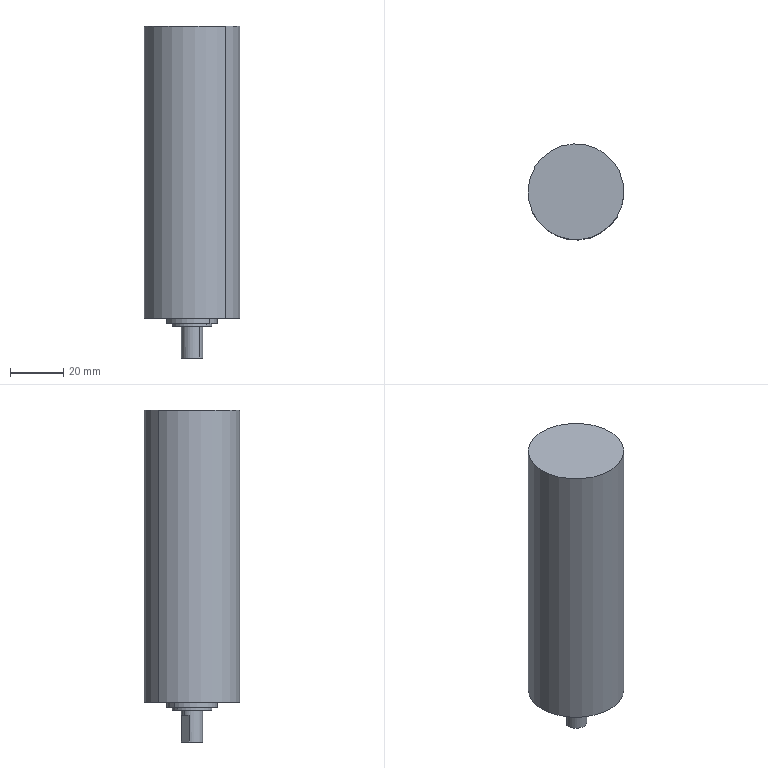Component | SolidWorks | MotorAssemblyWhen2-1_1.5KW-80-ER16A2-1 | 1 solid | 31 faces | box 36 x 36 x 124.7 mm | volume 112823 mm3 | cylinder 16 | cone 8 | plane 7 | commonest cylinder face diameters 2.5 x8 36 x2 19 x2 15 x2 8 x2
STEP:
#1=CARTESIAN_POINT('',(-1.467,4.834,0.5316));
#2=VERTEX_POINT('',#1);
#3=CARTESIAN_POINT('',(-2.47,5.836,0.5316));
#4=VERTEX_POINT('',#3);
#5=CARTESIAN_POINT('',(-1.969,5.335,0.5316));
#6=DIRECTION('',(-0.,0.,-1.));
#7=DIRECTION('',(0.7071,-0.7071,-0.));
#8=AXIS2_PLACEMENT_3D('',#5,#6,#7);
#9=CIRCLE('',#8,0.7087);
#10=EDGE_CURVE('',#2,#4,#9,.T.);
#11=ORIENTED_EDGE('',*,*,#10,.T.);
#12=CARTESIAN_POINT('',(-2.47,5.836,-3.787));
#13=VERTEX_POINT('',#12);
#14=CARTESIAN_POINT('',(-2.47,5.836,0.5316));
#15=DIRECTION('',(-0.,0.,-1.));
#16=VECTOR('',#15,39.37);
#17=LINE('',#14,#16);
#18=EDGE_CURVE('',#4,#13,#17,.T.);
#19=ORIENTED_EDGE('',*,*,#18,.T.);
#20=CARTESIAN_POINT('',(-1.467,4.834,-3.787));
#21=VERTEX_POINT('',#20);
#22=CARTESIAN_POINT('',(-1.969,5.335,-3.787));
#23=DIRECTION('',(0.,-0.,1.));
#24=DIRECTION('',(0.7071,-0.7071,0.));
#25=AXIS2_PLACEMENT_3D('',#22,#23,#24);
#26=CIRCLE('',#25,0.7087);
#27=EDGE_CURVE('',#13,#21,#26,.T.);
#28=ORIENTED_EDGE('',*,*,#27,.T.);
#29=CARTESIAN_POINT('',(-1.467,4.834,0.5316));
#30=DIRECTION('',(-0.,0.,-1.));
#31=VECTOR('',#30,39.37);
#32=LINE('',#29,#31);
#33=EDGE_CURVE('',#2,#21,#32,.T.);
#34=ORIENTED_EDGE('',*,*,#33,.F.);
#35=EDGE_LOOP('',(#11,#19,#28,#34));
#36=FACE_OUTER_BOUND('',#35,.T.);
#37=CARTESIAN_POINT('',(-1.969,5.335,0.5316));
#38=DIRECTION('',(-0.,0.,-1.));
#39=DIRECTION('',(0.7071,-0.7071,-0.));
#40=AXIS2_PLACEMENT_3D('',#37,#38,#39);
#41=CYLINDRICAL_SURFACE('',#40,0.7087);
#42=ADVANCED_FACE('',(#36),#41,.T.);
#43=CARTESIAN_POINT('',(-2.233,5.599,-3.866));
#44=VERTEX_POINT('',#43);
#45=CARTESIAN_POINT('',(-1.704,5.07,-3.866));
#46=VERTEX_POINT('',#45);
#47=CARTESIAN_POINT('',(-1.969,5.335,-3.866));
#48=DIRECTION('',(0.,-0.,1.));
#49=DIRECTION('',(-0.7071,0.7071,0.));
#50=AXIS2_PLACEMENT_3D('',#47,#48,#49);
#51=CIRCLE('',#50,0.374);
#52=EDGE_CURVE('',#44,#46,#51,.T.);
#53=ORIENTED_EDGE('',*,*,#52,.T.);
#54=CARTESIAN_POINT('',(-1.704,5.07,-3.787));
#55=VERTEX_POINT('',#54);
#56=CARTESIAN_POINT('',(-1.704,5.07,-3.866));
#57=DIRECTION('',(0.,-0.,1.));
#58=VECTOR('',#57,39.37);
#59=LINE('',#56,#58);
#60=EDGE_CURVE('',#46,#55,#59,.T.);
#61=ORIENTED_EDGE('',*,*,#60,.T.);
#62=CARTESIAN_POINT('',(-2.233,5.599,-3.787));
#63=VERTEX_POINT('',#62);
#64=CARTESIAN_POINT('',(-1.969,5.335,-3.787));
#65=DIRECTION('',(-0.,0.,-1.));
#66=DIRECTION('',(-0.7071,0.7071,0.));
#67=AXIS2_PLACEMENT_3D('',#64,#65,#66);
#68=CIRCLE('',#67,0.374);
#69=EDGE_CURVE('',#55,#63,#68,.T.);
#70=ORIENTED_EDGE('',*,*,#69,.T.);
#71=CARTESIAN_POINT('',(-2.233,5.599,-3.866));
#72=DIRECTION('',(0.,-0.,1.));
#73=VECTOR('',#72,39.37);
#74=LINE('',#71,#73);
#75=EDGE_CURVE('',#44,#63,#74,.T.);
#76=ORIENTED_EDGE('',*,*,#75,.F.);
#77=EDGE_LOOP('',(#53,#61,#70,#76));
#78=FACE_OUTER_BOUND('',#77,.T.);
#79=CARTESIAN_POINT('',(-1.969,5.335,-3.866));
#80=DIRECTION('',(0.,-0.,1.));
#81=DIRECTION('',(-0.7071,0.7071,0.));
#82=AXIS2_PLACEMENT_3D('',#79,#80,#81);
#83=CYLINDRICAL_SURFACE('',#82,0.374);
#84=ADVANCED_FACE('',(#78),#83,.T.);
#85=CARTESIAN_POINT('',(-2.435,4.938,-3.453));
#86=VERTEX_POINT('',#85);
#87=CARTESIAN_POINT('',(-2.365,4.868,-3.453));
#88=VERTEX_POINT('',#87);
#89=CARTESIAN_POINT('',(-2.4,4.903,-3.453));
#90=DIRECTION('',(-0.,0.,-1.));
#91=DIRECTION('',(0.7071,-0.7071,0.));
#92=AXIS2_PLACEMENT_3D('',#89,#90,#91);
#93=CIRCLE('',#92,0.04921);
#94=EDGE_CURVE('',#86,#88,#93,.T.);
#95=ORIENTED_EDGE('',*,*,#94,.F.);
#96=CARTESIAN_POINT('',(-2.435,4.938,-3.787));
#97=VERTEX_POINT('',#96);
#98=CARTESIAN_POINT('',(-2.435,4.938,-3.787));
#99=DIRECTION('',(-0.,0.,-1.));
#100=VECTOR('',#99,39.37);
#101=LINE('',#98,#100);
#102=EDGE_CURVE('',#86,#97,#101,.T.);
#103=ORIENTED_EDGE('',*,*,#102,.T.);
#104=CARTESIAN_POINT('',(-2.365,4.868,-3.787));
#105=VERTEX_POINT('',#104);
#106=CARTESIAN_POINT('',(-2.4,4.903,-3.787));
#107=DIRECTION('',(-0.,0.,-1.));
#108=DIRECTION('',(0.7071,-0.7071,0.));
#109=AXIS2_PLACEMENT_3D('',#106,#107,#108);
#110=CIRCLE('',#109,0.04921);
#111=EDGE_CURVE('',#97,#105,#110,.T.);
#112=ORIENTED_EDGE('',*,*,#111,.T.);
#113=CARTESIAN_POINT('',(-2.365,4.868,-3.787));
#114=DIRECTION('',(-0.,0.,-1.));
#115=VECTOR('',#114,39.37);
#116=LINE('',#113,#115);
#117=EDGE_CURVE('',#88,#105,#116,.T.);
#118=ORIENTED_EDGE('',*,*,#117,.F.);
#119=EDGE_LOOP('',(#95,#103,#112,#118));
#120=FACE_OUTER_BOUND('',#119,.T.);
#121=CARTESIAN_POINT('',(-2.4,4.903,-3.787));
#122=DIRECTION('',(-0.,0.,-1.));
#123=DIRECTION('',(0.7071,-0.7071,0.));
#124=AXIS2_PLACEMENT_3D('',#121,#122,#123);
#125=CYLINDRICAL_SURFACE('',#124,0.04921);
#126=ADVANCED_FACE('',(#120),#125,.F.);
#127=CARTESIAN_POINT('',(-1.572,4.938,-3.453));
#128=VERTEX_POINT('',#127);
#129=CARTESIAN_POINT('',(-1.502,4.868,-3.453));
#130=VERTEX_POINT('',#129);
#131=CARTESIAN_POINT('',(-1.537,4.903,-3.453));
#132=DIRECTION('',(-0.,0.,-1.));
#133=DIRECTION('',(0.7071,-0.7071,0.));
#134=AXIS2_PLACEMENT_3D('',#131,#132,#133);
#135=CIRCLE('',#134,0.04921);
#136=EDGE_CURVE('',#128,#130,#135,.T.);
#137=ORIENTED_EDGE('',*,*,#136,.F.);
#138=CARTESIAN_POINT('',(-1.572,4.938,-3.787));
#139=VERTEX_POINT('',#138);
#140=CARTESIAN_POINT('',(-1.572,4.938,-3.787));
#141=DIRECTION('',(-0.,0.,-1.));
#142=VECTOR('',#141,39.37);
#143=LINE('',#140,#142);
#144=EDGE_CURVE('',#128,#139,#143,.T.);
#145=ORIENTED_EDGE('',*,*,#144,.T.);
#146=CARTESIAN_POINT('',(-1.502,4.868,-3.787));
#147=VERTEX_POINT('',#146);
#148=CARTESIAN_POINT('',(-1.537,4.903,-3.787));
#149=DIRECTION('',(-0.,0.,-1.));
#150=DIRECTION('',(0.7071,-0.7071,0.));
#151=AXIS2_PLACEMENT_3D('',#148,#149,#150);
#152=CIRCLE('',#151,0.04921);
#153=EDGE_CURVE('',#139,#147,#152,.T.);
#154=ORIENTED_EDGE('',*,*,#153,.T.);
#155=CARTESIAN_POINT('',(-1.502,4.868,-3.787));
#156=DIRECTION('',(-0.,0.,-1.));
#157=VECTOR('',#156,39.37);
#158=LINE('',#155,#157);
#159=EDGE_CURVE('',#130,#147,#158,.T.);
#160=ORIENTED_EDGE('',*,*,#159,.F.);
#161=EDGE_LOOP('',(#137,#145,#154,#160));
#162=FACE_OUTER_BOUND('',#161,.T.);
#163=CARTESIAN_POINT('',(-1.537,4.903,-3.787));
#164=DIRECTION('',(-0.,0.,-1.));
#165=DIRECTION('',(0.7071,-0.7071,0.));
#166=AXIS2_PLACEMENT_3D('',#163,#164,#165);
#167=CYLINDRICAL_SURFACE('',#166,0.04921);
#168=ADVANCED_FACE('',(#162),#167,.F.);
#169=CARTESIAN_POINT('',(-1.572,5.801,-3.453));
#170=VERTEX_POINT('',#169);
#171=CARTESIAN_POINT('',(-1.502,5.731,-3.453));
#172=VERTEX_POINT('',#171);
#173=CARTESIAN_POINT('',(-1.537,5.766,-3.453));
#174=DIRECTION('',(-0.,0.,-1.));
#175=DIRECTION('',(0.7071,-0.7071,0.));
#176=AXIS2_PLACEMENT_3D('',#173,#174,#175);
#177=CIRCLE('',#176,0.04921);
#178=EDGE_CURVE('',#170,#172,#177,.T.);
#179=ORIENTED_EDGE('',*,*,#178,.F.);
#180=CARTESIAN_POINT('',(-1.572,5.801,-3.787));
#181=VERTEX_POINT('',#180);
#182=CARTESIAN_POINT('',(-1.572,5.801,-3.787));
#183=DIRECTION('',(-0.,0.,-1.));
#184=VECTOR('',#183,39.37);
#185=LINE('',#182,#184);
#186=EDGE_CURVE('',#170,#181,#185,.T.);
#187=ORIENTED_EDGE('',*,*,#186,.T.);
#188=CARTESIAN_POINT('',(-1.502,5.731,-3.787));
#189=VERTEX_POINT('',#188);
#190=CARTESIAN_POINT('',(-1.537,5.766,-3.787));
#191=DIRECTION('',(-0.,0.,-1.));
#192=DIRECTION('',(0.7071,-0.7071,0.));
#193=AXIS2_PLACEMENT_3D('',#190,#191,#192);
#194=CIRCLE('',#193,0.04921);
#195=EDGE_CURVE('',#181,#189,#194,.T.);
#196=ORIENTED_EDGE('',*,*,#195,.T.);
#197=CARTESIAN_POINT('',(-1.502,5.731,-3.787));
#198=DIRECTION('',(-0.,0.,-1.));
#199=VECTOR('',#198,39.37);
#200=LINE('',#197,#199);
#201=EDGE_CURVE('',#172,#189,#200,.T.);
#202=ORIENTED_EDGE('',*,*,#201,.F.);
#203=EDGE_LOOP('',(#179,#187,#196,#202));
#204=FACE_OUTER_BOUND('',#203,.T.);
#205=CARTESIAN_POINT('',(-1.537,5.766,-3.787));
#206=DIRECTION('',(-0.,0.,-1.));
#207=DIRECTION('',(0.7071,-0.7071,0.));
#208=AXIS2_PLACEMENT_3D('',#205,#206,#207);
#209=CYLINDRICAL_SURFACE('',#208,0.04921);
#210=ADVANCED_FACE('',(#204),#209,.F.);
#211=CARTESIAN_POINT('',(-2.435,5.801,-3.453));
#212=VERTEX_POINT('',#211);
#213=CARTESIAN_POINT('',(-2.365,5.731,-3.453));
#214=VERTEX_POINT('',#213);
#215=CARTESIAN_POINT('',(-2.4,5.766,-3.453));
#216=DIRECTION('',(-0.,0.,-1.));
#217=DIRECTION('',(0.7071,-0.7071,0.));
#218=AXIS2_PLACEMENT_3D('',#215,#216,#217);
#219=CIRCLE('',#218,0.04921);
#220=EDGE_CURVE('',#212,#214,#219,.T.);
#221=ORIENTED_EDGE('',*,*,#220,.F.);
#222=CARTESIAN_POINT('',(-2.435,5.801,-3.787));
#223=VERTEX_POINT('',#222);
#224=CARTESIAN_POINT('',(-2.435,5.801,-3.787));
#225=DIRECTION('',(-0.,0.,-1.));
#226=VECTOR('',#225,39.37);
#227=LINE('',#224,#226);
#228=EDGE_CURVE('',#212,#223,#227,.T.);
#229=ORIENTED_EDGE('',*,*,#228,.T.);
#230=CARTESIAN_POINT('',(-2.365,5.731,-3.787));
#231=VERTEX_POINT('',#230);
#232=CARTESIAN_POINT('',(-2.4,5.766,-3.787));
#233=DIRECTION('',(-0.,0.,-1.));
#234=DIRECTION('',(0.7071,-0.7071,0.));
#235=AXIS2_PLACEMENT_3D('',#232,#233,#234);
#236=CIRCLE('',#235,0.04921);
#237=EDGE_CURVE('',#223,#231,#236,.T.);
#238=ORIENTED_EDGE('',*,*,#237,.T.);
#239=CARTESIAN_POINT('',(-2.365,5.731,-3.787));
#240=DIRECTION('',(-0.,0.,-1.));
#241=VECTOR('',#240,39.37);
#242=LINE('',#239,#241);
#243=EDGE_CURVE('',#214,#231,#242,.T.);
#244=ORIENTED_EDGE('',*,*,#243,.F.);
#245=EDGE_LOOP('',(#221,#229,#238,#244));
#246=FACE_OUTER_BOUND('',#245,.T.);
#247=CARTESIAN_POINT('',(-2.4,5.766,-3.787));
#248=DIRECTION('',(-0.,0.,-1.));
#249=DIRECTION('',(0.7071,-0.7071,0.));
#250=AXIS2_PLACEMENT_3D('',#247,#248,#249);
#251=CYLINDRICAL_SURFACE('',#250,0.04921);
#252=ADVANCED_FACE('',(#246),#251,.F.);
#253=CARTESIAN_POINT('',(-2.4,4.903,-3.423));
#254=VERTEX_POINT('',#253);
#255=CARTESIAN_POINT('',(-2.365,4.868,-3.453));
#256=DIRECTION('',(0.6061,-0.6061,-0.515));
#257=VECTOR('',#256,39.37);
#258=LINE('',#255,#257);
#259=EDGE_CURVE('',#254,#88,#258,.T.);
#260=ORIENTED_EDGE('',*,*,#259,.F.);
#261=CARTESIAN_POINT('',(-2.435,4.938,-3.453));
#262=DIRECTION('',(-0.6061,0.6061,-0.515));
#263=VECTOR('',#262,39.37);
#264=LINE('',#261,#263);
#265=EDGE_CURVE('',#254,#86,#264,.T.);
#266=ORIENTED_EDGE('',*,*,#265,.T.);
#267=ORIENTED_EDGE('',*,*,#94,.T.);
#268=EDGE_LOOP('',(#260,#266,#267));
#269=FACE_OUTER_BOUND('',#268,.T.);
#270=CARTESIAN_POINT('',(-2.4,4.903,-3.453));
#271=DIRECTION('',(-0.,0.,-1.));
#272=DIRECTION('',(0.7071,-0.7071,0.));
#273=AXIS2_PLACEMENT_3D('',#270,#271,#272);
#274=CONICAL_SURFACE('',#273,0.04921,1.03);
#275=ADVANCED_FACE('',(#269),#274,.F.);
#276=CARTESIAN_POINT('',(-1.537,4.903,-3.423));
#277=VERTEX_POINT('',#276);
#278=CARTESIAN_POINT('',(-1.502,4.868,-3.453));
#279=DIRECTION('',(0.6061,-0.6061,-0.515));
#280=VECTOR('',#279,39.37);
#281=LINE('',#278,#280);
#282=EDGE_CURVE('',#277,#130,#281,.T.);
#283=ORIENTED_EDGE('',*,*,#282,.F.);
#284=CARTESIAN_POINT('',(-1.572,4.938,-3.453));
#285=DIRECTION('',(-0.6061,0.6061,-0.515));
#286=VECTOR('',#285,39.37);
#287=LINE('',#284,#286);
#288=EDGE_CURVE('',#277,#128,#287,.T.);
#289=ORIENTED_EDGE('',*,*,#288,.T.);
#290=ORIENTED_EDGE('',*,*,#136,.T.);
#291=EDGE_LOOP('',(#283,#289,#290));
#292=FACE_OUTER_BOUND('',#291,.T.);
#293=CARTESIAN_POINT('',(-1.537,4.903,-3.453));
#294=DIRECTION('',(-0.,0.,-1.));
#295=DIRECTION('',(0.7071,-0.7071,0.));
#296=AXIS2_PLACEMENT_3D('',#293,#294,#295);
#297=CONICAL_SURFACE('',#296,0.04921,1.03);
#298=ADVANCED_FACE('',(#292),#297,.F.);
#299=CARTESIAN_POINT('',(-1.537,5.766,-3.423));
#300=VERTEX_POINT('',#299);
#301=CARTESIAN_POINT('',(-1.502,5.731,-3.453));
#302=DIRECTION('',(0.6061,-0.6061,-0.515));
#303=VECTOR('',#302,39.37);
#304=LINE('',#301,#303);
#305=EDGE_CURVE('',#300,#172,#304,.T.);
#306=ORIENTED_EDGE('',*,*,#305,.F.);
#307=CARTESIAN_POINT('',(-1.572,5.801,-3.453));
#308=DIRECTION('',(-0.6061,0.6061,-0.515));
#309=VECTOR('',#308,39.37);
#310=LINE('',#307,#309);
#311=EDGE_CURVE('',#300,#170,#310,.T.);
#312=ORIENTED_EDGE('',*,*,#311,.T.);
#313=ORIENTED_EDGE('',*,*,#178,.T.);
#314=EDGE_LOOP('',(#306,#312,#313));
#315=FACE_OUTER_BOUND('',#314,.T.);
#316=CARTESIAN_POINT('',(-1.537,5.766,-3.453));
#317=DIRECTION('',(-0.,0.,-1.));
#318=DIRECTION('',(0.7071,-0.7071,0.));
#319=AXIS2_PLACEMENT_3D('',#316,#317,#318);
#320=CONICAL_SURFACE('',#319,0.04921,1.03);
#321=ADVANCED_FACE('',(#315),#320,.F.);
#322=CARTESIAN_POINT('',(-2.4,5.766,-3.423));
#323=VERTEX_POINT('',#322);
#324=CARTESIAN_POINT('',(-2.365,5.731,-3.453));
#325=DIRECTION('',(0.6061,-0.6061,-0.515));
#326=VECTOR('',#325,39.37);
#327=LINE('',#324,#326);
#328=EDGE_CURVE('',#323,#214,#327,.T.);
#329=ORIENTED_EDGE('',*,*,#328,.F.);
#330=CARTESIAN_POINT('',(-2.435,5.801,-3.453));
#331=DIRECTION('',(-0.6061,0.6061,-0.515));
#332=VECTOR('',#331,39.37);
#333=LINE('',#330,#332);
#334=EDGE_CURVE('',#323,#212,#333,.T.);
#335=ORIENTED_EDGE('',*,*,#334,.T.);
#336=ORIENTED_EDGE('',*,*,#220,.T.);
#337=EDGE_LOOP('',(#329,#335,#336));
#338=FACE_OUTER_BOUND('',#337,.T.);
#339=CARTESIAN_POINT('',(-2.4,5.766,-3.453));
#340=DIRECTION('',(-0.,0.,-1.));
#341=DIRECTION('',(0.7071,-0.7071,0.));
#342=AXIS2_PLACEMENT_3D('',#339,#340,#341);
#343=CONICAL_SURFACE('',#342,0.04921,1.03);
#344=ADVANCED_FACE('',(#338),#343,.F.);
#345=CARTESIAN_POINT('',(-2.177,5.543,-3.905));
#346=VERTEX_POINT('',#345);
#347=CARTESIAN_POINT('',(-1.76,5.126,-3.905));
#348=VERTEX_POINT('',#347);
#349=CARTESIAN_POINT('',(-1.969,5.335,-3.905));
#350=DIRECTION('',(0.,-0.,1.));
#351=DIRECTION('',(-0.7071,0.7071,0.));
#352=AXIS2_PLACEMENT_3D('',#349,#350,#351);
#353=CIRCLE('',#352,0.2953);
#354=EDGE_CURVE('',#346,#348,#353,.T.);
#355=ORIENTED_EDGE('',*,*,#354,.T.);
#356=CARTESIAN_POINT('',(-1.76,5.126,-3.866));
#357=VERTEX_POINT('',#356);
#358=CARTESIAN_POINT('',(-1.76,5.126,-3.905));
#359=DIRECTION('',(0.,-0.,1.));
#360=VECTOR('',#359,39.37);
#361=LINE('',#358,#360);
#362=EDGE_CURVE('',#348,#357,#361,.T.);
#363=ORIENTED_EDGE('',*,*,#362,.T.);
#364=CARTESIAN_POINT('',(-2.177,5.543,-3.866));
#365=VERTEX_POINT('',#364);
#366=CARTESIAN_POINT('',(-1.969,5.335,-3.866));
#367=DIRECTION('',(0.,-0.,1.));
#368=DIRECTION('',(-0.7071,0.7071,0.));
#369=AXIS2_PLACEMENT_3D('',#366,#367,#368);
#370=CIRCLE('',#369,0.2953);
#371=EDGE_CURVE('',#365,#357,#370,.T.);
#372=ORIENTED_EDGE('',*,*,#371,.F.);
#373=CARTESIAN_POINT('',(-2.177,5.543,-3.905));
#374=DIRECTION('',(0.,-0.,1.));
#375=VECTOR('',#374,39.37);
#376=LINE('',#373,#375);
#377=EDGE_CURVE('',#346,#365,#376,.T.);
#378=ORIENTED_EDGE('',*,*,#377,.F.);
#379=EDGE_LOOP('',(#355,#363,#372,#378));
#380=FACE_OUTER_BOUND('',#379,.T.);
#381=CARTESIAN_POINT('',(-1.969,5.335,-3.905));
#382=DIRECTION('',(0.,-0.,1.));
#383=DIRECTION('',(-0.7071,0.7071,0.));
#384=AXIS2_PLACEMENT_3D('',#381,#382,#383);
#385=CYLINDRICAL_SURFACE('',#384,0.2953);
#386=ADVANCED_FACE('',(#380),#385,.T.);
#387=CARTESIAN_POINT('',(-2.12,5.378,-4.378));
#388=VERTEX_POINT('',#387);
#389=CARTESIAN_POINT('',(-1.857,5.223,-4.378));
#390=VERTEX_POINT('',#389);
#391=CARTESIAN_POINT('',(-1.969,5.335,-4.378));
#392=DIRECTION('',(0.,-0.,1.));
#393=DIRECTION('',(-0.7071,0.7071,0.));
#394=AXIS2_PLACEMENT_3D('',#391,#392,#393);
#395=CIRCLE('',#394,0.1575);
#396=EDGE_CURVE('',#388,#390,#395,.T.);
#397=ORIENTED_EDGE('',*,*,#396,.T.);
#398=CARTESIAN_POINT('',(-1.857,5.223,-3.905));
#399=VERTEX_POINT('',#398);
#400=CARTESIAN_POINT('',(-1.857,5.223,-4.378));
#401=DIRECTION('',(0.,-0.,1.));
#402=VECTOR('',#401,39.37);
#403=LINE('',#400,#402);
#404=EDGE_CURVE('',#390,#399,#403,.T.);
#405=ORIENTED_EDGE('',*,*,#404,.T.);
#406=CARTESIAN_POINT('',(-2.08,5.446,-3.905));
#407=VERTEX_POINT('',#406);
#408=CARTESIAN_POINT('',(-1.969,5.335,-3.905));
#409=DIRECTION('',(0.,-0.,1.));
#410=DIRECTION('',(-0.7071,0.7071,0.));
#411=AXIS2_PLACEMENT_3D('',#408,#409,#410);
#412=CIRCLE('',#411,0.1575);
#413=EDGE_CURVE('',#407,#399,#412,.T.);
#414=ORIENTED_EDGE('',*,*,#413,.F.);
#415=CARTESIAN_POINT('',(-2.08,5.446,-3.984));
#416=VERTEX_POINT('',#415);
#417=CARTESIAN_POINT('',(-2.08,5.446,-4.378));
#418=DIRECTION('',(0.,-0.,1.));
#419=VECTOR('',#418,39.37);
#420=LINE('',#417,#419);
#421=EDGE_CURVE('',#416,#407,#420,.T.);
#422=ORIENTED_EDGE('',*,*,#421,.F.);
#423=CARTESIAN_POINT('',(-2.12,5.378,-3.984));
#424=VERTEX_POINT('',#423);
#425=CARTESIAN_POINT('',(-1.969,5.335,-3.984));
#426=DIRECTION('',(0.,-0.,1.));
#427=DIRECTION('',(-0.7071,0.7071,0.));
#428=AXIS2_PLACEMENT_3D('',#425,#426,#427);
#429=CIRCLE('',#428,0.1575);
#430=EDGE_CURVE('',#416,#424,#429,.T.);
#431=ORIENTED_EDGE('',*,*,#430,.T.);
#432=CARTESIAN_POINT('',(-2.12,5.378,-4.378));
#433=DIRECTION('',(-0.,0.,-1.));
#434=VECTOR('',#433,39.37);
#435=LINE('',#432,#434);
#436=EDGE_CURVE('',#424,#388,#435,.T.);
#437=ORIENTED_EDGE('',*,*,#436,.T.);
#438=EDGE_LOOP('',(#397,#405,#414,#422,#431,#437));
#439=FACE_OUTER_BOUND('',#438,.T.);
#440=CARTESIAN_POINT('',(-1.969,5.335,-4.378));
#441=DIRECTION('',(0.,-0.,1.));
#442=DIRECTION('',(-0.7071,0.7071,0.));
#443=AXIS2_PLACEMENT_3D('',#440,#441,#442);
#444=CYLINDRICAL_SURFACE('',#443,0.1575);
#445=ADVANCED_FACE('',(#439),#444,.T.);
#446=ORIENTED_EDGE('',*,*,#18,.F.);
#447=CARTESIAN_POINT('',(-1.969,5.335,0.5316));
#448=DIRECTION('',(-0.,0.,-1.));
#449=DIRECTION('',(0.7071,-0.7071,-0.));
#450=AXIS2_PLACEMENT_3D('',#447,#448,#449);
#451=CIRCLE('',#450,0.7087);
#452=EDGE_CURVE('',#4,#2,#451,.T.);
#453=ORIENTED_EDGE('',*,*,#452,.T.);
#454=ORIENTED_EDGE('',*,*,#33,.T.);
#455=CARTESIAN_POINT('',(-1.969,5.335,-3.787));
#456=DIRECTION('',(0.,-0.,1.));
#457=DIRECTION('',(0.7071,-0.7071,0.));
#458=AXIS2_PLACEMENT_3D('',#455,#456,#457);
#459=CIRCLE('',#458,0.7087);
#460=EDGE_CURVE('',#21,#13,#459,.T.);
#461=ORIENTED_EDGE('',*,*,#460,.T.);
#462=EDGE_LOOP('',(#446,#453,#454,#461));
#463=FACE_OUTER_BOUND('',#462,.T.);
#464=CARTESIAN_POINT('',(-1.969,5.335,0.5316));
#465=DIRECTION('',(-0.,0.,-1.));
#466=DIRECTION('',(0.7071,-0.7071,-0.));
#467=AXIS2_PLACEMENT_3D('',#464,#465,#466);
#468=CYLINDRICAL_SURFACE('',#467,0.7087);
#469=ADVANCED_FACE('',(#463),#468,.T.);
#470=CARTESIAN_POINT('',(-1.969,5.335,-3.787));
#471=DIRECTION('',(-0.,0.,-1.));
#472=DIRECTION('',(-0.7071,0.7071,0.));
#473=AXIS2_PLACEMENT_3D('',#470,#471,#472);
#474=CIRCLE('',#473,0.374);
#475=EDGE_CURVE('',#63,#55,#474,.T.);
#476=ORIENTED_EDGE('',*,*,#475,.F.);
#477=ORIENTED_EDGE('',*,*,#69,.F.);
#478=EDGE_LOOP('',(#476,#477));
#479=FACE_BOUND('',#478,.T.);
#480=ORIENTED_EDGE('',*,*,#460,.F.);
#481=ORIENTED_EDGE('',*,*,#27,.F.);
#482=EDGE_LOOP('',(#480,#481));
#483=FACE_OUTER_BOUND('',#482,.T.);
#484=CARTESIAN_POINT('',(-2.4,4.903,-3.787));
#485=DIRECTION('',(-0.,0.,-1.));
#486=DIRECTION('',(0.7071,-0.7071,0.));
#487=AXIS2_PLACEMENT_3D('',#484,#485,#486);
#488=CIRCLE('',#487,0.04921);
#489=EDGE_CURVE('',#105,#97,#488,.T.);
#490=ORIENTED_EDGE('',*,*,#489,.F.);
#491=ORIENTED_EDGE('',*,*,#111,.F.);
#492=EDGE_LOOP('',(#490,#491));
#493=FACE_BOUND('',#492,.T.);
#494=CARTESIAN_POINT('',(-1.537,4.903,-3.787));
#495=DIRECTION('',(-0.,0.,-1.));
#496=DIRECTION('',(0.7071,-0.7071,0.));
#497=AXIS2_PLACEMENT_3D('',#494,#495,#496);
#498=CIRCLE('',#497,0.04921);
#499=EDGE_CURVE('',#147,#139,#498,.T.);
#500=ORIENTED_EDGE('',*,*,#499,.F.);
#501=ORIENTED_EDGE('',*,*,#153,.F.);
#502=EDGE_LOOP('',(#500,#501));
#503=FACE_BOUND('',#502,.T.);
#504=CARTESIAN_POINT('',(-1.537,5.766,-3.787));
#505=DIRECTION('',(-0.,0.,-1.));
#506=DIRECTION('',(0.7071,-0.7071,0.));
#507=AXIS2_PLACEMENT_3D('',#504,#505,#506);
#508=CIRCLE('',#507,0.04921);
#509=EDGE_CURVE('',#189,#181,#508,.T.);
#510=ORIENTED_EDGE('',*,*,#509,.F.);
#511=ORIENTED_EDGE('',*,*,#195,.F.);
#512=EDGE_LOOP('',(#510,#511));
#513=FACE_BOUND('',#512,.T.);
#514=CARTESIAN_POINT('',(-2.4,5.766,-3.787));
#515=DIRECTION('',(-0.,0.,-1.));
#516=DIRECTION('',(0.7071,-0.7071,0.));
#517=AXIS2_PLACEMENT_3D('',#514,#515,#516);
#518=CIRCLE('',#517,0.04921);
#519=EDGE_CURVE('',#231,#223,#518,.T.);
#520=ORIENTED_EDGE('',*,*,#519,.F.);
#521=ORIENTED_EDGE('',*,*,#237,.F.);
#522=EDGE_LOOP('',(#520,#521));
#523=FACE_BOUND('',#522,.T.);
#524=CARTESIAN_POINT('',(-1.969,5.335,-3.787));
#525=DIRECTION('',(0.,-0.,1.));
#526=DIRECTION('',(-0.7071,0.7071,0.));
#527=AXIS2_PLACEMENT_3D('',#524,#525,#526);
#528=PLANE('',#527);
#529=ADVANCED_FACE('',(#479,#483,#493,#503,#513,#523),#528,.F.);
#530=ORIENTED_EDGE('',*,*,#10,.F.);
#531=ORIENTED_EDGE('',*,*,#452,.F.);
#532=EDGE_LOOP('',(#530,#531));
#533=FACE_OUTER_BOUND('',#532,.T.);
#534=CARTESIAN_POINT('',(-1.969,5.335,0.5316));
#535=DIRECTION('',(0.,-0.,1.));
#536=DIRECTION('',(-0.7071,0.7071,0.));
#537=AXIS2_PLACEMENT_3D('',#534,#535,#536);
#538=PLANE('',#537);
#539=ADVANCED_FACE('',(#533),#538,.T.);
#540=ORIENTED_EDGE('',*,*,#60,.F.);
#541=CARTESIAN_POINT('',(-1.969,5.335,-3.866));
#542=DIRECTION('',(0.,-0.,1.));
#543=DIRECTION('',(-0.7071,0.7071,0.));
#544=AXIS2_PLACEMENT_3D('',#541,#542,#543);
#545=CIRCLE('',#544,0.374);
#546=EDGE_CURVE('',#46,#44,#545,.T.);
#547=ORIENTED_EDGE('',*,*,#546,.T.);
#548=ORIENTED_EDGE('',*,*,#75,.T.);
#549=ORIENTED_EDGE('',*,*,#475,.T.);
#550=EDGE_LOOP('',(#540,#547,#548,#549));
#551=FACE_OUTER_BOUND('',#550,.T.);
#552=CARTESIAN_POINT('',(-1.969,5.335,-3.866));
#553=DIRECTION('',(0.,-0.,1.));
#554=DIRECTION('',(-0.7071,0.7071,0.));
#555=AXIS2_PLACEMENT_3D('',#552,#553,#554);
#556=CYLINDRICAL_SURFACE('',#555,0.374);
#557=ADVANCED_FACE('',(#551),#556,.T.);
#558=ORIENTED_EDGE('',*,*,#102,.F.);
#559=CARTESIAN_POINT('',(-2.4,4.903,-3.453));
#560=DIRECTION('',(-0.,0.,-1.));
#561=DIRECTION('',(0.7071,-0.7071,0.));
#562=AXIS2_PLACEMENT_3D('',#559,#560,#561);
#563=CIRCLE('',#562,0.04921);
#564=EDGE_CURVE('',#88,#86,#563,.T.);
#565=ORIENTED_EDGE('',*,*,#564,.F.);
#566=ORIENTED_EDGE('',*,*,#117,.T.);
#567=ORIENTED_EDGE('',*,*,#489,.T.);
#568=EDGE_LOOP('',(#558,#565,#566,#567));
#569=FACE_OUTER_BOUND('',#568,.T.);
#570=CARTESIAN_POINT('',(-2.4,4.903,-3.787));
#571=DIRECTION('',(-0.,0.,-1.));
#572=DIRECTION('',(0.7071,-0.7071,0.));
#573=AXIS2_PLACEMENT_3D('',#570,#571,#572);
#574=CYLINDRICAL_SURFACE('',#573,0.04921);
#575=ADVANCED_FACE('',(#569),#574,.F.);
#576=ORIENTED_EDGE('',*,*,#144,.F.);
#577=CARTESIAN_POINT('',(-1.537,4.903,-3.453));
#578=DIRECTION('',(-0.,0.,-1.));
#579=DIRECTION('',(0.7071,-0.7071,0.));
#580=AXIS2_PLACEMENT_3D('',#577,#578,#579);
#581=CIRCLE('',#580,0.04921);
#582=EDGE_CURVE('',#130,#128,#581,.T.);
#583=ORIENTED_EDGE('',*,*,#582,.F.);
#584=ORIENTED_EDGE('',*,*,#159,.T.);
#585=ORIENTED_EDGE('',*,*,#499,.T.);
#586=EDGE_LOOP('',(#576,#583,#584,#585));
#587=FACE_OUTER_BOUND('',#586,.T.);
#588=CARTESIAN_POINT('',(-1.537,4.903,-3.787));
#589=DIRECTION('',(-0.,0.,-1.));
#590=DIRECTION('',(0.7071,-0.7071,0.));
#591=AXIS2_PLACEMENT_3D('',#588,#589,#590);
#592=CYLINDRICAL_SURFACE('',#591,0.04921);
#593=ADVANCED_FACE('',(#587),#592,.F.);
#594=ORIENTED_EDGE('',*,*,#186,.F.);
#595=CARTESIAN_POINT('',(-1.537,5.766,-3.453));
#596=DIRECTION('',(-0.,0.,-1.));
#597=DIRECTION('',(0.7071,-0.7071,0.));
#598=AXIS2_PLACEMENT_3D('',#595,#596,#597);
#599=CIRCLE('',#598,0.04921);
#600=EDGE_CURVE('',#172,#170,#599,.T.);
#601=ORIENTED_EDGE('',*,*,#600,.F.);
#602=ORIENTED_EDGE('',*,*,#201,.T.);
#603=ORIENTED_EDGE('',*,*,#509,.T.);
#604=EDGE_LOOP('',(#594,#601,#602,#603));
#605=FACE_OUTER_BOUND('',#604,.T.);
#606=CARTESIAN_POINT('',(-1.537,5.766,-3.787));
#607=DIRECTION('',(-0.,0.,-1.));
#608=DIRECTION('',(0.7071,-0.7071,0.));
#609=AXIS2_PLACEMENT_3D('',#606,#607,#608);
#610=CYLINDRICAL_SURFACE('',#609,0.04921);
#611=ADVANCED_FACE('',(#605),#610,.F.);
#612=ORIENTED_EDGE('',*,*,#228,.F.);
#613=CARTESIAN_POINT('',(-2.4,5.766,-3.453));
#614=DIRECTION('',(-0.,0.,-1.));
#615=DIRECTION('',(0.7071,-0.7071,0.));
#616=AXIS2_PLACEMENT_3D('',#613,#614,#615);
#617=CIRCLE('',#616,0.04921);
#618=EDGE_CURVE('',#214,#212,#617,.T.);
#619=ORIENTED_EDGE('',*,*,#618,.F.);
#620=ORIENTED_EDGE('',*,*,#243,.T.);
#621=ORIENTED_EDGE('',*,*,#519,.T.);
#622=EDGE_LOOP('',(#612,#619,#620,#621));
#623=FACE_OUTER_BOUND('',#622,.T.);
#624=CARTESIAN_POINT('',(-2.4,5.766,-3.787));
#625=DIRECTION('',(-0.,0.,-1.));
#626=DIRECTION('',(0.7071,-0.7071,0.));
#627=AXIS2_PLACEMENT_3D('',#624,#625,#626);
#628=CYLINDRICAL_SURFACE('',#627,0.04921);
#629=ADVANCED_FACE('',(#623),#628,.F.);
#630=ORIENTED_EDGE('',*,*,#371,.T.);
#631=CARTESIAN_POINT('',(-1.969,5.335,-3.866));
#632=DIRECTION('',(0.,-0.,1.));
#633=DIRECTION('',(-0.7071,0.7071,0.));
#634=AXIS2_PLACEMENT_3D('',#631,#632,#633);
#635=CIRCLE('',#634,0.2953);
#636=EDGE_CURVE('',#357,#365,#635,.T.);
#637=ORIENTED_EDGE('',*,*,#636,.T.);
#638=EDGE_LOOP('',(#630,#637));
#639=FACE_BOUND('',#638,.T.);
#640=ORIENTED_EDGE('',*,*,#52,.F.);
#641=ORIENTED_EDGE('',*,*,#546,.F.);
#642=EDGE_LOOP('',(#640,#641));
#643=FACE_OUTER_BOUND('',#642,.T.);
#644=CARTESIAN_POINT('',(-1.969,5.335,-3.866));
#645=DIRECTION('',(-0.,0.,-1.));
#646=DIRECTION('',(0.7071,-0.7071,-0.));
#647=AXIS2_PLACEMENT_3D('',#644,#645,#646);
#648=PLANE('',#647);
#649=ADVANCED_FACE('',(#639,#643),#648,.T.);
#650=ORIENTED_EDGE('',*,*,#265,.F.);
#651=ORIENTED_EDGE('',*,*,#259,.T.);
#652=ORIENTED_EDGE('',*,*,#564,.T.);
#653=EDGE_LOOP('',(#650,#651,#652));
#654=FACE_OUTER_BOUND('',#653,.T.);
#655=CARTESIAN_POINT('',(-2.4,4.903,-3.453));
#656=DIRECTION('',(-0.,0.,-1.));
#657=DIRECTION('',(0.7071,-0.7071,0.));
#658=AXIS2_PLACEMENT_3D('',#655,#656,#657);
#659=CONICAL_SURFACE('',#658,0.04921,1.03);
#660=ADVANCED_FACE('',(#654),#659,.F.);
#661=ORIENTED_EDGE('',*,*,#288,.F.);
#662=ORIENTED_EDGE('',*,*,#282,.T.);
#663=ORIENTED_EDGE('',*,*,#582,.T.);
#664=EDGE_LOOP('',(#661,#662,#663));
#665=FACE_OUTER_BOUND('',#664,.T.);
#666=CARTESIAN_POINT('',(-1.537,4.903,-3.453));
#667=DIRECTION('',(-0.,0.,-1.));
#668=DIRECTION('',(0.7071,-0.7071,0.));
#669=AXIS2_PLACEMENT_3D('',#666,#667,#668);
#670=CONICAL_SURFACE('',#669,0.04921,1.03);
#671=ADVANCED_FACE('',(#665),#670,.F.);
#672=ORIENTED_EDGE('',*,*,#311,.F.);
#673=ORIENTED_EDGE('',*,*,#305,.T.);
#674=ORIENTED_EDGE('',*,*,#600,.T.);
#675=EDGE_LOOP('',(#672,#673,#674));
#676=FACE_OUTER_BOUND('',#675,.T.);
#677=CARTESIAN_POINT('',(-1.537,5.766,-3.453));
#678=DIRECTION('',(-0.,0.,-1.));
#679=DIRECTION('',(0.7071,-0.7071,0.));
#680=AXIS2_PLACEMENT_3D('',#677,#678,#679);
#681=CONICAL_SURFACE('',#680,0.04921,1.03);
#682=ADVANCED_FACE('',(#676),#681,.F.);
#683=ORIENTED_EDGE('',*,*,#334,.F.);
#684=ORIENTED_EDGE('',*,*,#328,.T.);
#685=ORIENTED_EDGE('',*,*,#618,.T.);
#686=EDGE_LOOP('',(#683,#684,#685));
#687=FACE_OUTER_BOUND('',#686,.T.);
#688=CARTESIAN_POINT('',(-2.4,5.766,-3.453));
#689=DIRECTION('',(-0.,0.,-1.));
#690=DIRECTION('',(0.7071,-0.7071,0.));
#691=AXIS2_PLACEMENT_3D('',#688,#689,#690);
#692=CONICAL_SURFACE('',#691,0.04921,1.03);
#693=ADVANCED_FACE('',(#687),#692,.F.);
#694=ORIENTED_EDGE('',*,*,#362,.F.);
#695=CARTESIAN_POINT('',(-1.969,5.335,-3.905));
#696=DIRECTION('',(0.,-0.,1.));
#697=DIRECTION('',(-0.7071,0.7071,0.));
#698=AXIS2_PLACEMENT_3D('',#695,#696,#697);
#699=CIRCLE('',#698,0.2953);
#700=EDGE_CURVE('',#348,#346,#699,.T.);
#701=ORIENTED_EDGE('',*,*,#700,.T.);
#702=ORIENTED_EDGE('',*,*,#377,.T.);
#703=ORIENTED_EDGE('',*,*,#636,.F.);
#704=EDGE_LOOP('',(#694,#701,#702,#703));
#705=FACE_OUTER_BOUND('',#704,.T.);
#706=CARTESIAN_POINT('',(-1.969,5.335,-3.905));
#707=DIRECTION('',(0.,-0.,1.));
#708=DIRECTION('',(-0.7071,0.7071,0.));
#709=AXIS2_PLACEMENT_3D('',#706,#707,#708);
#710=CYLINDRICAL_SURFACE('',#709,0.2953);
#711=ADVANCED_FACE('',(#705),#710,.T.);
#712=ORIENTED_EDGE('',*,*,#413,.T.);
#713=CARTESIAN_POINT('',(-1.969,5.335,-3.905));
#714=DIRECTION('',(0.,-0.,1.));
#715=DIRECTION('',(-0.7071,0.7071,0.));
#716=AXIS2_PLACEMENT_3D('',#713,#714,#715);
#717=CIRCLE('',#716,0.1575);
#718=EDGE_CURVE('',#399,#407,#717,.T.);
#719=ORIENTED_EDGE('',*,*,#718,.T.);
#720=EDGE_LOOP('',(#712,#719));
#721=FACE_BOUND('',#720,.T.);
#722=ORIENTED_EDGE('',*,*,#354,.F.);
#723=ORIENTED_EDGE('',*,*,#700,.F.);
#724=EDGE_LOOP('',(#722,#723));
#725=FACE_OUTER_BOUND('',#724,.T.);
#726=CARTESIAN_POINT('',(-1.969,5.335,-3.905));
#727=DIRECTION('',(-0.,0.,-1.));
#728=DIRECTION('',(0.7071,-0.7071,-0.));
#729=AXIS2_PLACEMENT_3D('',#726,#727,#728);
#730=PLANE('',#729);
#731=ADVANCED_FACE('',(#721,#725),#730,.T.);
#732=ORIENTED_EDGE('',*,*,#404,.F.);
#733=CARTESIAN_POINT('',(-2.012,5.486,-4.378));
#734=VERTEX_POINT('',#733);
#735=CARTESIAN_POINT('',(-1.969,5.335,-4.378));
#736=DIRECTION('',(0.,-0.,1.));
#737=DIRECTION('',(-0.7071,0.7071,0.));
#738=AXIS2_PLACEMENT_3D('',#735,#736,#737);
#739=CIRCLE('',#738,0.1575);
#740=EDGE_CURVE('',#390,#734,#739,.T.);
#741=ORIENTED_EDGE('',*,*,#740,.T.);
#742=CARTESIAN_POINT('',(-2.012,5.486,-3.984));
#743=VERTEX_POINT('',#742);
#744=CARTESIAN_POINT('',(-2.012,5.486,-4.378));
#745=DIRECTION('',(0.,-0.,1.));
#746=VECTOR('',#745,39.37);
#747=LINE('',#744,#746);
#748=EDGE_CURVE('',#734,#743,#747,.T.);
#749=ORIENTED_EDGE('',*,*,#748,.T.);
#750=CARTESIAN_POINT('',(-1.969,5.335,-3.984));
#751=DIRECTION('',(0.,-0.,1.));
#752=DIRECTION('',(-0.7071,0.7071,0.));
#753=AXIS2_PLACEMENT_3D('',#750,#751,#752);
#754=CIRCLE('',#753,0.1575);
#755=EDGE_CURVE('',#743,#416,#754,.T.);
#756=ORIENTED_EDGE('',*,*,#755,.T.);
#757=ORIENTED_EDGE('',*,*,#421,.T.);
#758=ORIENTED_EDGE('',*,*,#718,.F.);
#759=EDGE_LOOP('',(#732,#741,#749,#756,#757,#758));
#760=FACE_OUTER_BOUND('',#759,.T.);
#761=CARTESIAN_POINT('',(-1.969,5.335,-4.378));
#762=DIRECTION('',(0.,-0.,1.));
#763=DIRECTION('',(-0.7071,0.7071,0.));
#764=AXIS2_PLACEMENT_3D('',#761,#762,#763);
#765=CYLINDRICAL_SURFACE('',#764,0.1575);
#766=ADVANCED_FACE('',(#760),#765,.T.);
#767=ORIENTED_EDGE('',*,*,#436,.F.);
#768=CARTESIAN_POINT('',(-1.951,5.547,-3.984));
#769=DIRECTION('',(-0.7071,-0.7071,-0.));
#770=VECTOR('',#769,39.37);
#771=LINE('',#768,#770);
#772=EDGE_CURVE('',#743,#424,#771,.T.);
#773=ORIENTED_EDGE('',*,*,#772,.F.);
#774=ORIENTED_EDGE('',*,*,#748,.F.);
#775=CARTESIAN_POINT('',(-1.951,5.547,-4.378));
#776=DIRECTION('',(0.7071,0.7071,0.));
#777=VECTOR('',#776,39.37);
#778=LINE('',#775,#777);
#779=EDGE_CURVE('',#388,#734,#778,.T.);
#780=ORIENTED_EDGE('',*,*,#779,.F.);
#781=EDGE_LOOP('',(#767,#773,#774,#780));
#782=FACE_OUTER_BOUND('',#781,.T.);
#783=CARTESIAN_POINT('',(-1.951,5.547,-3.984));
#784=DIRECTION('',(0.7071,-0.7071,-0.));
#785=DIRECTION('',(0.7071,0.7071,0.));
#786=AXIS2_PLACEMENT_3D('',#783,#784,#785);
#787=PLANE('',#786);
#788=ADVANCED_FACE('',(#782),#787,.F.);
#789=ORIENTED_EDGE('',*,*,#755,.F.);
#790=ORIENTED_EDGE('',*,*,#772,.T.);
#791=ORIENTED_EDGE('',*,*,#430,.F.);
#792=EDGE_LOOP('',(#789,#790,#791));
#793=FACE_OUTER_BOUND('',#792,.T.);
#794=CARTESIAN_POINT('',(-1.969,5.335,-3.984));
#795=DIRECTION('',(-0.,0.,-1.));
#796=DIRECTION('',(0.7071,-0.7071,-0.));
#797=AXIS2_PLACEMENT_3D('',#794,#795,#796);
#798=PLANE('',#797);
#799=ADVANCED_FACE('',(#793),#798,.T.);
#800=ORIENTED_EDGE('',*,*,#779,.T.);
#801=ORIENTED_EDGE('',*,*,#740,.F.);
#802=ORIENTED_EDGE('',*,*,#396,.F.);
#803=EDGE_LOOP('',(#800,#801,#802));
#804=FACE_OUTER_BOUND('',#803,.T.);
#805=CARTESIAN_POINT('',(-1.969,5.335,-4.378));
#806=DIRECTION('',(-0.,0.,-1.));
#807=DIRECTION('',(0.7071,-0.7071,-0.));
#808=AXIS2_PLACEMENT_3D('',#805,#806,#807);
#809=PLANE('',#808);
#810=ADVANCED_FACE('',(#804),#809,.T.);
#811=CLOSED_SHELL('',(#42,#84,#126,#168,#210,#252,#275,#298,#321,#344,#386,#445,#469,#529,#539,#557,#575,#593,#611,#629,#649,#660,#671,#682,#693,#711,#731,#766,#788,#799,#810));
#812=MANIFOLD_SOLID_BREP('',#811);
#813=CARTESIAN_POINT('',(0.,0.,0.));
#814=DIRECTION('',(0.,0.,1.));
#815=DIRECTION('',(1.,0.,0.));
#816=AXIS2_PLACEMENT_3D('',#813,#814,#815);
#817=(LENGTH_UNIT()NAMED_UNIT(*)SI_UNIT($,.METRE.));
#818=LENGTH_MEASURE_WITH_UNIT(LENGTH_MEASURE(0.0254),#817);
#819=DIMENSIONAL_EXPONENTS(1.,0.,0.,0.,0.,0.,0.);
#820=(CONVERSION_BASED_UNIT('',#818)LENGTH_UNIT()NAMED_UNIT(#819));
#821=UNCERTAINTY_MEASURE_WITH_UNIT(LENGTH_MEASURE(0.00001),#820,'','');
#822=(NAMED_UNIT(*)PLANE_ANGLE_UNIT()SI_UNIT($,.RADIAN.));
#823=(NAMED_UNIT(*)SI_UNIT($,.STERADIAN.)SOLID_ANGLE_UNIT());
#824=(GEOMETRIC_REPRESENTATION_CONTEXT(3)GLOBAL_UNCERTAINTY_ASSIGNED_CONTEXT((#821))GLOBAL_UNIT_ASSIGNED_CONTEXT((#820,#822,#823))REPRESENTATION_CONTEXT('',''));
#825=ADVANCED_BREP_SHAPE_REPRESENTATION('',(#812,#816),#824);
#826=COLOUR_RGB('',0.7922,0.8196,0.9333);
#827=FILL_AREA_STYLE_COLOUR('',#826);
#828=FILL_AREA_STYLE('',(#827));
#829=SURFACE_STYLE_FILL_AREA(#828);
#830=SURFACE_SIDE_STYLE('',(#829));
#831=SURFACE_STYLE_USAGE(.BOTH.,#830);
#832=PRESENTATION_STYLE_ASSIGNMENT((#831));
#833=STYLED_ITEM('',(#832),#812);
#834=PRESENTATION_LAYER_ASSIGNMENT('','',(#833));
#835=(LENGTH_UNIT()NAMED_UNIT(*)SI_UNIT($,.METRE.));
#836=LENGTH_MEASURE_WITH_UNIT(LENGTH_MEASURE(0.0254),#835);
#837=DIMENSIONAL_EXPONENTS(1.,0.,0.,0.,0.,0.,0.);
#838=(CONVERSION_BASED_UNIT('',#836)LENGTH_UNIT()NAMED_UNIT(#837));
#839=UNCERTAINTY_MEASURE_WITH_UNIT(LENGTH_MEASURE(0.00001),#838,'','');
#840=(NAMED_UNIT(*)PLANE_ANGLE_UNIT()SI_UNIT($,.RADIAN.));
#841=(NAMED_UNIT(*)SI_UNIT($,.STERADIAN.)SOLID_ANGLE_UNIT());
#842=(GEOMETRIC_REPRESENTATION_CONTEXT(3)GLOBAL_UNCERTAINTY_ASSIGNED_CONTEXT((#839))GLOBAL_UNIT_ASSIGNED_CONTEXT((#838,#840,#841))REPRESENTATION_CONTEXT('',''));
#843=MECHANICAL_DESIGN_GEOMETRIC_PRESENTATION_REPRESENTATION('',(#833),#842);